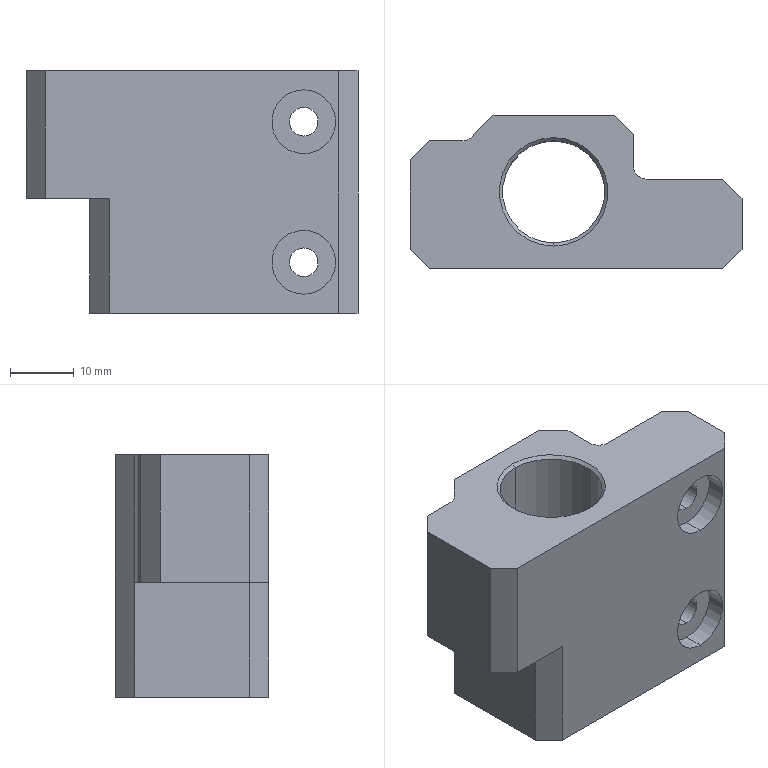Component | SolidWorks | DZ.KX.203-TC1505-30-09-01-05-10-1 | 1 solid | 42 faces | volume 26185 mm3 | plane 22 | cylinder 16 | cone 4 | commonest cylinder face diameters 7.5 x4 4.5 x4 10 x4 16 x2 4 x2 | material Plain Carbon Steel